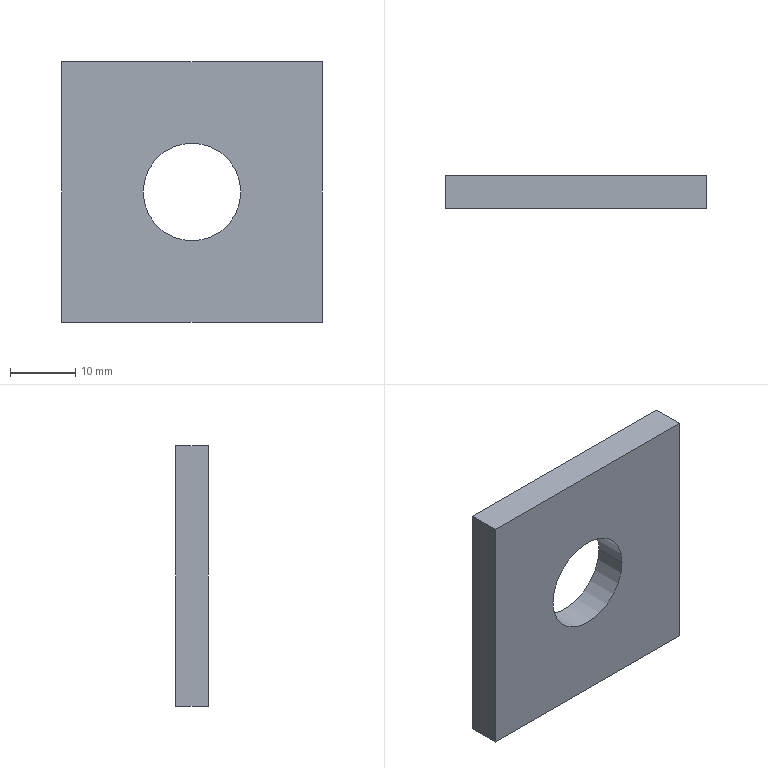Component | SolidWorks | MotorAxisHousingBase2-2 | 1 solid | 8 faces | box 40 x 5 x 40 mm | volume 7116 mm3 | plane 6 | cylinder 2 | commonest cylinder face diameters 15 x2
build123d program:
from build123d import *

# Parameters (mm, degrees)
SKETCH1_W           = 40
SKETCH1_H           = 40
SKETCH1_R           = 7.5
BOSS_EXTRUDE1_DEPTH = 5


with BuildPart() as part:
    # Sketch1 → Boss-Extrude1 (new body)
    with BuildSketch(Plane.XY):
        with Locations((-296.282, -20)):
            Rectangle(SKETCH1_W, SKETCH1_H)
        with Locations((-296.282, -20)):
            Circle(SKETCH1_R, mode=Mode.SUBTRACT)
    extrude(amount=BOSS_EXTRUDE1_DEPTH)


solid = part.part

# Placed as in the assembly
solid = solid.moved(Location((259.282, 200, 26), (90, 0, 0)))
STEP:
#1=CARTESIAN_POINT('',(-1.752,7.874,0.2362));
#2=VERTEX_POINT('',#1);
#3=CARTESIAN_POINT('',(-1.161,7.874,0.2362));
#4=VERTEX_POINT('',#3);
#5=CARTESIAN_POINT('',(-1.457,7.874,0.2362));
#6=DIRECTION('',(0.,1.,0.));
#7=DIRECTION('',(1.,0.,0.));
#8=AXIS2_PLACEMENT_3D('',#5,#6,#7);
#9=CIRCLE('',#8,0.2953);
#10=EDGE_CURVE('',#2,#4,#9,.T.);
#11=ORIENTED_EDGE('',*,*,#10,.T.);
#12=CARTESIAN_POINT('',(-1.161,7.677,0.2362));
#13=VERTEX_POINT('',#12);
#14=CARTESIAN_POINT('',(-1.161,7.874,0.2362));
#15=DIRECTION('',(0.,-1.,0.));
#16=VECTOR('',#15,39.37);
#17=LINE('',#14,#16);
#18=EDGE_CURVE('',#4,#13,#17,.T.);
#19=ORIENTED_EDGE('',*,*,#18,.T.);
#20=CARTESIAN_POINT('',(-1.752,7.677,0.2362));
#21=VERTEX_POINT('',#20);
#22=CARTESIAN_POINT('',(-1.457,7.677,0.2362));
#23=DIRECTION('',(0.,1.,0.));
#24=DIRECTION('',(1.,0.,0.));
#25=AXIS2_PLACEMENT_3D('',#22,#23,#24);
#26=CIRCLE('',#25,0.2953);
#27=EDGE_CURVE('',#21,#13,#26,.T.);
#28=ORIENTED_EDGE('',*,*,#27,.F.);
#29=CARTESIAN_POINT('',(-1.752,7.874,0.2362));
#30=DIRECTION('',(0.,-1.,0.));
#31=VECTOR('',#30,39.37);
#32=LINE('',#29,#31);
#33=EDGE_CURVE('',#2,#21,#32,.T.);
#34=ORIENTED_EDGE('',*,*,#33,.F.);
#35=EDGE_LOOP('',(#11,#19,#28,#34));
#36=FACE_OUTER_BOUND('',#35,.T.);
#37=CARTESIAN_POINT('',(-1.457,7.874,0.2362));
#38=DIRECTION('',(0.,-1.,0.));
#39=DIRECTION('',(-1.,0.,0.));
#40=AXIS2_PLACEMENT_3D('',#37,#38,#39);
#41=CYLINDRICAL_SURFACE('',#40,0.2953);
#42=ADVANCED_FACE('',(#36),#41,.F.);
#43=CARTESIAN_POINT('',(-2.244,7.874,-0.5512));
#44=VERTEX_POINT('',#43);
#45=CARTESIAN_POINT('',(-2.244,7.874,1.024));
#46=VERTEX_POINT('',#45);
#47=CARTESIAN_POINT('',(-2.244,7.874,1.024));
#48=DIRECTION('',(0.,0.,1.));
#49=VECTOR('',#48,39.37);
#50=LINE('',#47,#49);
#51=EDGE_CURVE('',#44,#46,#50,.T.);
#52=ORIENTED_EDGE('',*,*,#51,.T.);
#53=CARTESIAN_POINT('',(-0.6693,7.874,1.024));
#54=VERTEX_POINT('',#53);
#55=CARTESIAN_POINT('',(-0.6693,7.874,1.024));
#56=DIRECTION('',(1.,0.,-0.));
#57=VECTOR('',#56,39.37);
#58=LINE('',#55,#57);
#59=EDGE_CURVE('',#46,#54,#58,.T.);
#60=ORIENTED_EDGE('',*,*,#59,.T.);
#61=CARTESIAN_POINT('',(-0.6693,7.874,-0.5512));
#62=VERTEX_POINT('',#61);
#63=CARTESIAN_POINT('',(-0.6693,7.874,1.024));
#64=DIRECTION('',(0.,0.,-1.));
#65=VECTOR('',#64,39.37);
#66=LINE('',#63,#65);
#67=EDGE_CURVE('',#54,#62,#66,.T.);
#68=ORIENTED_EDGE('',*,*,#67,.T.);
#69=CARTESIAN_POINT('',(-0.6693,7.874,-0.5512));
#70=DIRECTION('',(-1.,0.,0.));
#71=VECTOR('',#70,39.37);
#72=LINE('',#69,#71);
#73=EDGE_CURVE('',#62,#44,#72,.T.);
#74=ORIENTED_EDGE('',*,*,#73,.T.);
#75=EDGE_LOOP('',(#52,#60,#68,#74));
#76=FACE_OUTER_BOUND('',#75,.T.);
#77=ORIENTED_EDGE('',*,*,#10,.F.);
#78=CARTESIAN_POINT('',(-1.457,7.874,0.2362));
#79=DIRECTION('',(0.,1.,0.));
#80=DIRECTION('',(1.,0.,0.));
#81=AXIS2_PLACEMENT_3D('',#78,#79,#80);
#82=CIRCLE('',#81,0.2953);
#83=EDGE_CURVE('',#4,#2,#82,.T.);
#84=ORIENTED_EDGE('',*,*,#83,.F.);
#85=EDGE_LOOP('',(#77,#84));
#86=FACE_BOUND('',#85,.T.);
#87=CARTESIAN_POINT('',(10.208,7.874,-0.5512));
#88=DIRECTION('',(0.,1.,0.));
#89=DIRECTION('',(1.,0.,0.));
#90=AXIS2_PLACEMENT_3D('',#87,#88,#89);
#91=PLANE('',#90);
#92=ADVANCED_FACE('',(#76,#86),#91,.T.);
#93=CARTESIAN_POINT('',(-2.244,7.677,-0.5512));
#94=VERTEX_POINT('',#93);
#95=CARTESIAN_POINT('',(-2.244,7.677,1.024));
#96=VERTEX_POINT('',#95);
#97=CARTESIAN_POINT('',(-2.244,7.677,1.024));
#98=DIRECTION('',(0.,0.,1.));
#99=VECTOR('',#98,39.37);
#100=LINE('',#97,#99);
#101=EDGE_CURVE('',#94,#96,#100,.T.);
#102=ORIENTED_EDGE('',*,*,#101,.F.);
#103=CARTESIAN_POINT('',(-0.6693,7.677,-0.5512));
#104=VERTEX_POINT('',#103);
#105=CARTESIAN_POINT('',(-0.6693,7.677,-0.5512));
#106=DIRECTION('',(-1.,0.,0.));
#107=VECTOR('',#106,39.37);
#108=LINE('',#105,#107);
#109=EDGE_CURVE('',#104,#94,#108,.T.);
#110=ORIENTED_EDGE('',*,*,#109,.F.);
#111=CARTESIAN_POINT('',(-0.6693,7.677,1.024));
#112=VERTEX_POINT('',#111);
#113=CARTESIAN_POINT('',(-0.6693,7.677,1.024));
#114=DIRECTION('',(0.,0.,-1.));
#115=VECTOR('',#114,39.37);
#116=LINE('',#113,#115);
#117=EDGE_CURVE('',#112,#104,#116,.T.);
#118=ORIENTED_EDGE('',*,*,#117,.F.);
#119=CARTESIAN_POINT('',(-0.6693,7.677,1.024));
#120=DIRECTION('',(1.,0.,-0.));
#121=VECTOR('',#120,39.37);
#122=LINE('',#119,#121);
#123=EDGE_CURVE('',#96,#112,#122,.T.);
#124=ORIENTED_EDGE('',*,*,#123,.F.);
#125=EDGE_LOOP('',(#102,#110,#118,#124));
#126=FACE_OUTER_BOUND('',#125,.T.);
#127=ORIENTED_EDGE('',*,*,#27,.T.);
#128=CARTESIAN_POINT('',(-1.457,7.677,0.2362));
#129=DIRECTION('',(0.,1.,0.));
#130=DIRECTION('',(1.,0.,0.));
#131=AXIS2_PLACEMENT_3D('',#128,#129,#130);
#132=CIRCLE('',#131,0.2953);
#133=EDGE_CURVE('',#13,#21,#132,.T.);
#134=ORIENTED_EDGE('',*,*,#133,.T.);
#135=EDGE_LOOP('',(#127,#134));
#136=FACE_BOUND('',#135,.T.);
#137=CARTESIAN_POINT('',(10.208,7.677,-0.5512));
#138=DIRECTION('',(0.,1.,0.));
#139=DIRECTION('',(1.,0.,0.));
#140=AXIS2_PLACEMENT_3D('',#137,#138,#139);
#141=PLANE('',#140);
#142=ADVANCED_FACE('',(#126,#136),#141,.F.);
#143=ORIENTED_EDGE('',*,*,#101,.T.);
#144=CARTESIAN_POINT('',(-2.244,7.874,1.024));
#145=DIRECTION('',(0.,-1.,0.));
#146=VECTOR('',#145,39.37);
#147=LINE('',#144,#146);
#148=EDGE_CURVE('',#46,#96,#147,.T.);
#149=ORIENTED_EDGE('',*,*,#148,.F.);
#150=ORIENTED_EDGE('',*,*,#51,.F.);
#151=CARTESIAN_POINT('',(-2.244,7.874,-0.5512));
#152=DIRECTION('',(0.,-1.,0.));
#153=VECTOR('',#152,39.37);
#154=LINE('',#151,#153);
#155=EDGE_CURVE('',#44,#94,#154,.T.);
#156=ORIENTED_EDGE('',*,*,#155,.T.);
#157=EDGE_LOOP('',(#143,#149,#150,#156));
#158=FACE_OUTER_BOUND('',#157,.T.);
#159=CARTESIAN_POINT('',(-2.244,7.874,1.024));
#160=DIRECTION('',(1.,0.,-0.));
#161=DIRECTION('',(-0.,0.,-1.));
#162=AXIS2_PLACEMENT_3D('',#159,#160,#161);
#163=PLANE('',#162);
#164=ADVANCED_FACE('',(#158),#163,.F.);
#165=ORIENTED_EDGE('',*,*,#123,.T.);
#166=CARTESIAN_POINT('',(-0.6693,7.874,1.024));
#167=DIRECTION('',(0.,-1.,0.));
#168=VECTOR('',#167,39.37);
#169=LINE('',#166,#168);
#170=EDGE_CURVE('',#54,#112,#169,.T.);
#171=ORIENTED_EDGE('',*,*,#170,.F.);
#172=ORIENTED_EDGE('',*,*,#59,.F.);
#173=ORIENTED_EDGE('',*,*,#148,.T.);
#174=EDGE_LOOP('',(#165,#171,#172,#173));
#175=FACE_OUTER_BOUND('',#174,.T.);
#176=CARTESIAN_POINT('',(-0.6693,7.874,1.024));
#177=DIRECTION('',(-0.,0.,-1.));
#178=DIRECTION('',(-1.,0.,0.));
#179=AXIS2_PLACEMENT_3D('',#176,#177,#178);
#180=PLANE('',#179);
#181=ADVANCED_FACE('',(#175),#180,.F.);
#182=ORIENTED_EDGE('',*,*,#117,.T.);
#183=CARTESIAN_POINT('',(-0.6693,7.874,-0.5512));
#184=DIRECTION('',(0.,-1.,0.));
#185=VECTOR('',#184,39.37);
#186=LINE('',#183,#185);
#187=EDGE_CURVE('',#62,#104,#186,.T.);
#188=ORIENTED_EDGE('',*,*,#187,.F.);
#189=ORIENTED_EDGE('',*,*,#67,.F.);
#190=ORIENTED_EDGE('',*,*,#170,.T.);
#191=EDGE_LOOP('',(#182,#188,#189,#190));
#192=FACE_OUTER_BOUND('',#191,.T.);
#193=CARTESIAN_POINT('',(-0.6693,7.874,1.024));
#194=DIRECTION('',(-1.,0.,0.));
#195=DIRECTION('',(0.,1.,0.));
#196=AXIS2_PLACEMENT_3D('',#193,#194,#195);
#197=PLANE('',#196);
#198=ADVANCED_FACE('',(#192),#197,.F.);
#199=ORIENTED_EDGE('',*,*,#109,.T.);
#200=ORIENTED_EDGE('',*,*,#155,.F.);
#201=ORIENTED_EDGE('',*,*,#73,.F.);
#202=ORIENTED_EDGE('',*,*,#187,.T.);
#203=EDGE_LOOP('',(#199,#200,#201,#202));
#204=FACE_OUTER_BOUND('',#203,.T.);
#205=CARTESIAN_POINT('',(-0.6693,7.874,-0.5512));
#206=DIRECTION('',(0.,0.,1.));
#207=DIRECTION('',(0.,-1.,0.));
#208=AXIS2_PLACEMENT_3D('',#205,#206,#207);
#209=PLANE('',#208);
#210=ADVANCED_FACE('',(#204),#209,.F.);
#211=ORIENTED_EDGE('',*,*,#18,.F.);
#212=ORIENTED_EDGE('',*,*,#83,.T.);
#213=ORIENTED_EDGE('',*,*,#33,.T.);
#214=ORIENTED_EDGE('',*,*,#133,.F.);
#215=EDGE_LOOP('',(#211,#212,#213,#214));
#216=FACE_OUTER_BOUND('',#215,.T.);
#217=CARTESIAN_POINT('',(-1.457,7.874,0.2362));
#218=DIRECTION('',(0.,-1.,0.));
#219=DIRECTION('',(-1.,0.,0.));
#220=AXIS2_PLACEMENT_3D('',#217,#218,#219);
#221=CYLINDRICAL_SURFACE('',#220,0.2953);
#222=ADVANCED_FACE('',(#216),#221,.F.);
#223=CLOSED_SHELL('',(#42,#92,#142,#164,#181,#198,#210,#222));
#224=MANIFOLD_SOLID_BREP('',#223);
#225=CARTESIAN_POINT('',(0.,0.,0.));
#226=DIRECTION('',(0.,0.,1.));
#227=DIRECTION('',(1.,0.,0.));
#228=AXIS2_PLACEMENT_3D('',#225,#226,#227);
#229=(LENGTH_UNIT()NAMED_UNIT(*)SI_UNIT($,.METRE.));
#230=LENGTH_MEASURE_WITH_UNIT(LENGTH_MEASURE(0.0254),#229);
#231=DIMENSIONAL_EXPONENTS(1.,0.,0.,0.,0.,0.,0.);
#232=(CONVERSION_BASED_UNIT('',#230)LENGTH_UNIT()NAMED_UNIT(#231));
#233=UNCERTAINTY_MEASURE_WITH_UNIT(LENGTH_MEASURE(0.00001),#232,'','');
#234=(NAMED_UNIT(*)PLANE_ANGLE_UNIT()SI_UNIT($,.RADIAN.));
#235=(NAMED_UNIT(*)SI_UNIT($,.STERADIAN.)SOLID_ANGLE_UNIT());
#236=(GEOMETRIC_REPRESENTATION_CONTEXT(3)GLOBAL_UNCERTAINTY_ASSIGNED_CONTEXT((#233))GLOBAL_UNIT_ASSIGNED_CONTEXT((#232,#234,#235))REPRESENTATION_CONTEXT('',''));
#237=ADVANCED_BREP_SHAPE_REPRESENTATION('',(#224,#228),#236);
#238=COLOUR_RGB('',0.7922,0.8196,0.9333);
#239=FILL_AREA_STYLE_COLOUR('',#238);
#240=FILL_AREA_STYLE('',(#239));
#241=SURFACE_STYLE_FILL_AREA(#240);
#242=SURFACE_SIDE_STYLE('',(#241));
#243=SURFACE_STYLE_USAGE(.BOTH.,#242);
#244=PRESENTATION_STYLE_ASSIGNMENT((#243));
#245=STYLED_ITEM('',(#244),#224);
#246=(LENGTH_UNIT()NAMED_UNIT(*)SI_UNIT($,.METRE.));
#247=LENGTH_MEASURE_WITH_UNIT(LENGTH_MEASURE(0.0254),#246);
#248=DIMENSIONAL_EXPONENTS(1.,0.,0.,0.,0.,0.,0.);
#249=(CONVERSION_BASED_UNIT('',#247)LENGTH_UNIT()NAMED_UNIT(#248));
#250=UNCERTAINTY_MEASURE_WITH_UNIT(LENGTH_MEASURE(0.00001),#249,'','');
#251=(NAMED_UNIT(*)PLANE_ANGLE_UNIT()SI_UNIT($,.RADIAN.));
#252=(NAMED_UNIT(*)SI_UNIT($,.STERADIAN.)SOLID_ANGLE_UNIT());
#253=(GEOMETRIC_REPRESENTATION_CONTEXT(3)GLOBAL_UNCERTAINTY_ASSIGNED_CONTEXT((#250))GLOBAL_UNIT_ASSIGNED_CONTEXT((#249,#251,#252))REPRESENTATION_CONTEXT('',''));
#254=MECHANICAL_DESIGN_GEOMETRIC_PRESENTATION_REPRESENTATION('',(#245),#253);
#255=PRESENTATION_LAYER_ASSIGNMENT('','',(#245));